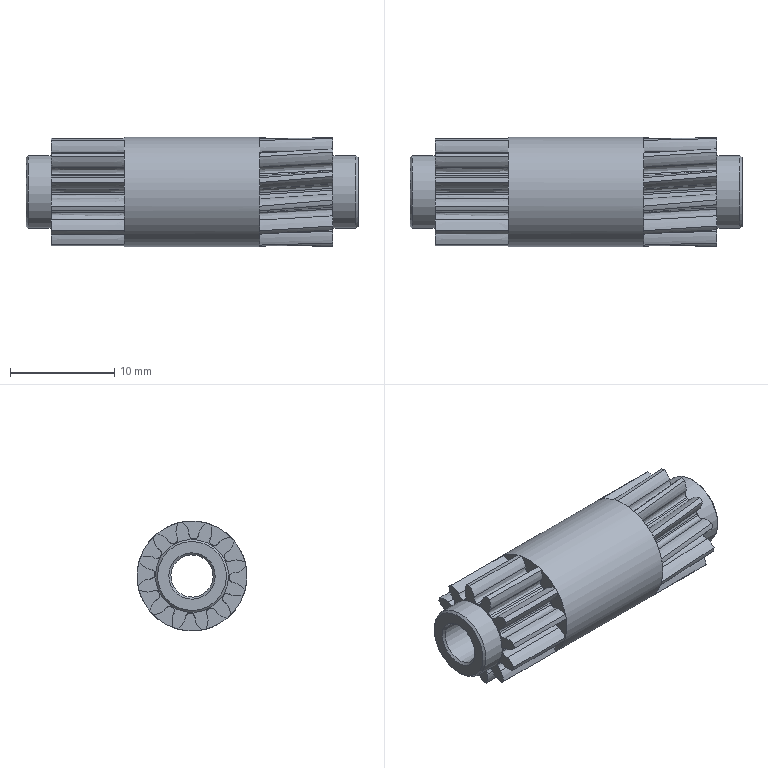Component | NX | DJZ_07_WORM_GEAR | 1 solid | 191 faces | volume 1762 mm3 | other 60 | spline 60 | plane 40 | cylinder 28 | cone 3 | commonest cylinder face diameters 7.125 x12 7.15 x12 7 x2 10.5 x1 4.05 x1